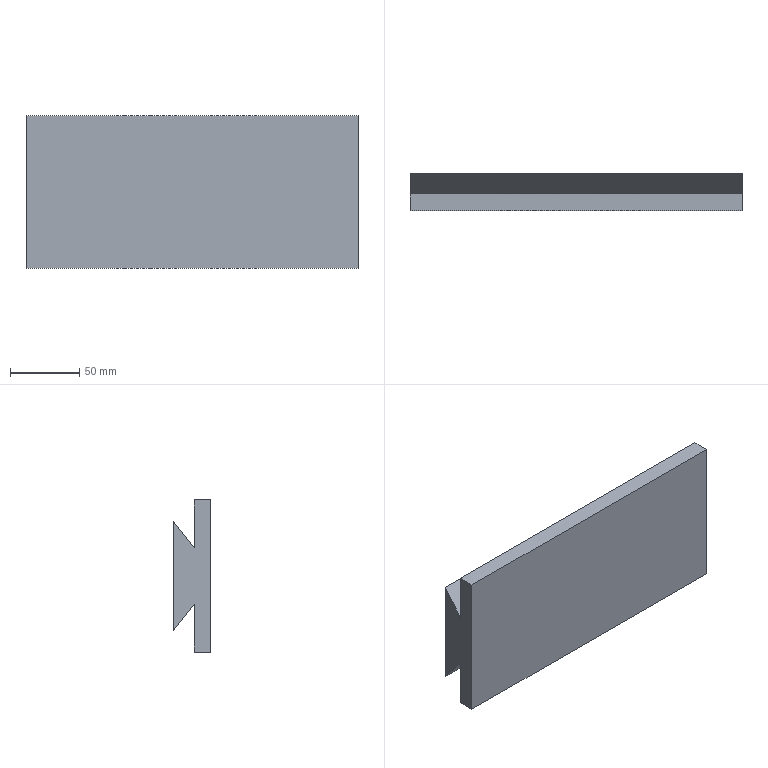Component | SolidWorks | PassiveRollerAssembly-1_DovetailPlate-1 | 1 solid | 10 faces | box 240 x 27 x 110 mm | volume 532800 mm3 | plane 10
build123d program:
from build123d import *

# Parameters (mm, degrees)
BOSS_EXTRUDE1_DEPTH = 240


with BuildPart() as part:
    # Sketch1 → Boss-Extrude1 (new body)
    with BuildSketch(Plane.XY):
        Polygon((-55, 0), (55, 0), (55, 12), (20.5, 12), (39.5, 27), (-39.5, 27), (-20.5, 12), (-55, 12), align=None)
    extrude(amount=BOSS_EXTRUDE1_DEPTH)


solid = part.part

# Placed as in the assembly
solid = solid.moved(Location((2085, 550, 270), (0, 90, 0)))
STEP:
#1=COLOUR_RGB('',0.7922,0.8196,0.9333);
#2=FILL_AREA_STYLE_COLOUR('',#1);
#3=FILL_AREA_STYLE('',(#2));
#4=SURFACE_STYLE_FILL_AREA(#3);
#5=SURFACE_SIDE_STYLE('',(#4));
#6=SURFACE_STYLE_USAGE(.BOTH.,#5);
#7=PRESENTATION_STYLE_ASSIGNMENT((#6));
#8=CARTESIAN_POINT('',(82.087,21.654,8.465));
#9=VERTEX_POINT('',#8);
#10=CARTESIAN_POINT('',(82.087,22.126,8.465));
#11=VERTEX_POINT('',#10);
#12=CARTESIAN_POINT('',(82.087,21.654,8.465));
#13=DIRECTION('',(0.,1.,-0.));
#14=VECTOR('',#13,39.37);
#15=LINE('',#12,#14);
#16=EDGE_CURVE('',#9,#11,#15,.T.);
#17=ORIENTED_EDGE('',*,*,#16,.T.);
#18=CARTESIAN_POINT('',(91.535,22.126,8.465));
#19=VERTEX_POINT('',#18);
#20=CARTESIAN_POINT('',(91.535,22.126,8.465));
#21=DIRECTION('',(-1.,0.,0.));
#22=VECTOR('',#21,39.37);
#23=LINE('',#20,#22);
#24=EDGE_CURVE('',#19,#11,#23,.T.);
#25=ORIENTED_EDGE('',*,*,#24,.F.);
#26=CARTESIAN_POINT('',(91.535,21.654,8.465));
#27=VERTEX_POINT('',#26);
#28=CARTESIAN_POINT('',(91.535,21.654,8.465));
#29=DIRECTION('',(0.,1.,-0.));
#30=VECTOR('',#29,39.37);
#31=LINE('',#28,#30);
#32=EDGE_CURVE('',#27,#19,#31,.T.);
#33=ORIENTED_EDGE('',*,*,#32,.F.);
#34=CARTESIAN_POINT('',(91.535,21.654,8.465));
#35=DIRECTION('',(-1.,0.,0.));
#36=VECTOR('',#35,39.37);
#37=LINE('',#34,#36);
#38=EDGE_CURVE('',#27,#9,#37,.T.);
#39=ORIENTED_EDGE('',*,*,#38,.T.);
#40=EDGE_LOOP('',(#17,#25,#33,#39));
#41=FACE_OUTER_BOUND('',#40,.T.);
#42=CARTESIAN_POINT('',(91.535,21.654,8.465));
#43=DIRECTION('',(0.,0.,1.));
#44=DIRECTION('',(0.,-1.,0.));
#45=AXIS2_PLACEMENT_3D('',#42,#43,#44);
#46=PLANE('',#45);
#47=ADVANCED_FACE('',(#41),#46,.F.);
#48=CARTESIAN_POINT('',(82.087,22.126,9.823));
#49=VERTEX_POINT('',#48);
#50=CARTESIAN_POINT('',(82.087,22.126,8.465));
#51=DIRECTION('',(0.,-0.,1.));
#52=VECTOR('',#51,39.37);
#53=LINE('',#50,#52);
#54=EDGE_CURVE('',#11,#49,#53,.T.);
#55=ORIENTED_EDGE('',*,*,#54,.T.);
#56=CARTESIAN_POINT('',(91.535,22.126,9.823));
#57=VERTEX_POINT('',#56);
#58=CARTESIAN_POINT('',(91.535,22.126,9.823));
#59=DIRECTION('',(-1.,0.,0.));
#60=VECTOR('',#59,39.37);
#61=LINE('',#58,#60);
#62=EDGE_CURVE('',#57,#49,#61,.T.);
#63=ORIENTED_EDGE('',*,*,#62,.F.);
#64=CARTESIAN_POINT('',(91.535,22.126,8.465));
#65=DIRECTION('',(0.,-0.,1.));
#66=VECTOR('',#65,39.37);
#67=LINE('',#64,#66);
#68=EDGE_CURVE('',#19,#57,#67,.T.);
#69=ORIENTED_EDGE('',*,*,#68,.F.);
#70=ORIENTED_EDGE('',*,*,#24,.T.);
#71=EDGE_LOOP('',(#55,#63,#69,#70));
#72=FACE_OUTER_BOUND('',#71,.T.);
#73=CARTESIAN_POINT('',(91.535,22.126,8.465));
#74=DIRECTION('',(0.,-1.,-0.));
#75=DIRECTION('',(0.,0.,-1.));
#76=AXIS2_PLACEMENT_3D('',#73,#74,#75);
#77=PLANE('',#76);
#78=ADVANCED_FACE('',(#72),#77,.F.);
#79=CARTESIAN_POINT('',(82.087,22.717,9.075));
#80=VERTEX_POINT('',#79);
#81=CARTESIAN_POINT('',(82.087,22.126,9.823));
#82=DIRECTION('',(0.,0.6196,-0.7849));
#83=VECTOR('',#82,39.37);
#84=LINE('',#81,#83);
#85=EDGE_CURVE('',#49,#80,#84,.T.);
#86=ORIENTED_EDGE('',*,*,#85,.T.);
#87=CARTESIAN_POINT('',(91.535,22.717,9.075));
#88=VERTEX_POINT('',#87);
#89=CARTESIAN_POINT('',(91.535,22.717,9.075));
#90=DIRECTION('',(-1.,0.,0.));
#91=VECTOR('',#90,39.37);
#92=LINE('',#89,#91);
#93=EDGE_CURVE('',#88,#80,#92,.T.);
#94=ORIENTED_EDGE('',*,*,#93,.F.);
#95=CARTESIAN_POINT('',(91.535,22.126,9.823));
#96=DIRECTION('',(0.,0.6196,-0.7849));
#97=VECTOR('',#96,39.37);
#98=LINE('',#95,#97);
#99=EDGE_CURVE('',#57,#88,#98,.T.);
#100=ORIENTED_EDGE('',*,*,#99,.F.);
#101=ORIENTED_EDGE('',*,*,#62,.T.);
#102=EDGE_LOOP('',(#86,#94,#100,#101));
#103=FACE_OUTER_BOUND('',#102,.T.);
#104=CARTESIAN_POINT('',(91.535,22.126,9.823));
#105=DIRECTION('',(0.,0.7849,0.6196));
#106=DIRECTION('',(0.,-0.6196,0.7849));
#107=AXIS2_PLACEMENT_3D('',#104,#105,#106);
#108=PLANE('',#107);
#109=ADVANCED_FACE('',(#103),#108,.F.);
#110=CARTESIAN_POINT('',(82.087,22.717,12.185));
#111=VERTEX_POINT('',#110);
#112=CARTESIAN_POINT('',(82.087,22.717,9.075));
#113=DIRECTION('',(0.,-0.,1.));
#114=VECTOR('',#113,39.37);
#115=LINE('',#112,#114);
#116=EDGE_CURVE('',#80,#111,#115,.T.);
#117=ORIENTED_EDGE('',*,*,#116,.T.);
#118=CARTESIAN_POINT('',(91.535,22.717,12.185));
#119=VERTEX_POINT('',#118);
#120=CARTESIAN_POINT('',(91.535,22.717,12.185));
#121=DIRECTION('',(-1.,0.,0.));
#122=VECTOR('',#121,39.37);
#123=LINE('',#120,#122);
#124=EDGE_CURVE('',#119,#111,#123,.T.);
#125=ORIENTED_EDGE('',*,*,#124,.F.);
#126=CARTESIAN_POINT('',(91.535,22.717,9.075));
#127=DIRECTION('',(0.,-0.,1.));
#128=VECTOR('',#127,39.37);
#129=LINE('',#126,#128);
#130=EDGE_CURVE('',#88,#119,#129,.T.);
#131=ORIENTED_EDGE('',*,*,#130,.F.);
#132=ORIENTED_EDGE('',*,*,#93,.T.);
#133=EDGE_LOOP('',(#117,#125,#131,#132));
#134=FACE_OUTER_BOUND('',#133,.T.);
#135=CARTESIAN_POINT('',(91.535,22.717,9.075));
#136=DIRECTION('',(0.,-1.,-0.));
#137=DIRECTION('',(0.,0.,-1.));
#138=AXIS2_PLACEMENT_3D('',#135,#136,#137);
#139=PLANE('',#138);
#140=ADVANCED_FACE('',(#134),#139,.F.);
#141=CARTESIAN_POINT('',(82.087,22.126,11.437));
#142=VERTEX_POINT('',#141);
#143=CARTESIAN_POINT('',(82.087,22.126,11.437));
#144=DIRECTION('',(0.,-0.6196,-0.7849));
#145=VECTOR('',#144,39.37);
#146=LINE('',#143,#145);
#147=EDGE_CURVE('',#111,#142,#146,.T.);
#148=ORIENTED_EDGE('',*,*,#147,.T.);
#149=CARTESIAN_POINT('',(91.535,22.126,11.437));
#150=VERTEX_POINT('',#149);
#151=CARTESIAN_POINT('',(91.535,22.126,11.437));
#152=DIRECTION('',(-1.,0.,0.));
#153=VECTOR('',#152,39.37);
#154=LINE('',#151,#153);
#155=EDGE_CURVE('',#150,#142,#154,.T.);
#156=ORIENTED_EDGE('',*,*,#155,.F.);
#157=CARTESIAN_POINT('',(91.535,22.126,11.437));
#158=DIRECTION('',(0.,-0.6196,-0.7849));
#159=VECTOR('',#158,39.37);
#160=LINE('',#157,#159);
#161=EDGE_CURVE('',#119,#150,#160,.T.);
#162=ORIENTED_EDGE('',*,*,#161,.F.);
#163=ORIENTED_EDGE('',*,*,#124,.T.);
#164=EDGE_LOOP('',(#148,#156,#162,#163));
#165=FACE_OUTER_BOUND('',#164,.T.);
#166=CARTESIAN_POINT('',(91.535,22.126,11.437));
#167=DIRECTION('',(0.,0.7849,-0.6196));
#168=DIRECTION('',(0.,0.6196,0.7849));
#169=AXIS2_PLACEMENT_3D('',#166,#167,#168);
#170=PLANE('',#169);
#171=ADVANCED_FACE('',(#165),#170,.F.);
#172=CARTESIAN_POINT('',(82.087,22.126,12.795));
#173=VERTEX_POINT('',#172);
#174=CARTESIAN_POINT('',(82.087,22.126,12.795));
#175=DIRECTION('',(0.,0.,1.));
#176=VECTOR('',#175,39.37);
#177=LINE('',#174,#176);
#178=EDGE_CURVE('',#142,#173,#177,.T.);
#179=ORIENTED_EDGE('',*,*,#178,.T.);
#180=CARTESIAN_POINT('',(91.535,22.126,12.795));
#181=VERTEX_POINT('',#180);
#182=CARTESIAN_POINT('',(91.535,22.126,12.795));
#183=DIRECTION('',(-1.,0.,0.));
#184=VECTOR('',#183,39.37);
#185=LINE('',#182,#184);
#186=EDGE_CURVE('',#181,#173,#185,.T.);
#187=ORIENTED_EDGE('',*,*,#186,.F.);
#188=CARTESIAN_POINT('',(91.535,22.126,12.795));
#189=DIRECTION('',(0.,0.,1.));
#190=VECTOR('',#189,39.37);
#191=LINE('',#188,#190);
#192=EDGE_CURVE('',#150,#181,#191,.T.);
#193=ORIENTED_EDGE('',*,*,#192,.F.);
#194=ORIENTED_EDGE('',*,*,#155,.T.);
#195=EDGE_LOOP('',(#179,#187,#193,#194));
#196=FACE_OUTER_BOUND('',#195,.T.);
#197=CARTESIAN_POINT('',(91.535,22.126,12.795));
#198=DIRECTION('',(0.,-1.,0.));
#199=DIRECTION('',(0.,-0.,-1.));
#200=AXIS2_PLACEMENT_3D('',#197,#198,#199);
#201=PLANE('',#200);
#202=ADVANCED_FACE('',(#196),#201,.F.);
#203=CARTESIAN_POINT('',(82.087,21.654,12.795));
#204=VERTEX_POINT('',#203);
#205=CARTESIAN_POINT('',(82.087,21.654,12.795));
#206=DIRECTION('',(0.,-1.,-0.));
#207=VECTOR('',#206,39.37);
#208=LINE('',#205,#207);
#209=EDGE_CURVE('',#173,#204,#208,.T.);
#210=ORIENTED_EDGE('',*,*,#209,.T.);
#211=CARTESIAN_POINT('',(91.535,21.654,12.795));
#212=VERTEX_POINT('',#211);
#213=CARTESIAN_POINT('',(91.535,21.654,12.795));
#214=DIRECTION('',(-1.,0.,0.));
#215=VECTOR('',#214,39.37);
#216=LINE('',#213,#215);
#217=EDGE_CURVE('',#212,#204,#216,.T.);
#218=ORIENTED_EDGE('',*,*,#217,.F.);
#219=CARTESIAN_POINT('',(91.535,21.654,12.795));
#220=DIRECTION('',(0.,-1.,-0.));
#221=VECTOR('',#220,39.37);
#222=LINE('',#219,#221);
#223=EDGE_CURVE('',#181,#212,#222,.T.);
#224=ORIENTED_EDGE('',*,*,#223,.F.);
#225=ORIENTED_EDGE('',*,*,#186,.T.);
#226=EDGE_LOOP('',(#210,#218,#224,#225));
#227=FACE_OUTER_BOUND('',#226,.T.);
#228=CARTESIAN_POINT('',(91.535,21.654,12.795));
#229=DIRECTION('',(0.,0.,-1.));
#230=DIRECTION('',(0.,1.,0.));
#231=AXIS2_PLACEMENT_3D('',#228,#229,#230);
#232=PLANE('',#231);
#233=ADVANCED_FACE('',(#227),#232,.F.);
#234=CARTESIAN_POINT('',(82.087,21.654,12.795));
#235=DIRECTION('',(0.,0.,-1.));
#236=VECTOR('',#235,39.37);
#237=LINE('',#234,#236);
#238=EDGE_CURVE('',#204,#9,#237,.T.);
#239=ORIENTED_EDGE('',*,*,#238,.T.);
#240=ORIENTED_EDGE('',*,*,#38,.F.);
#241=CARTESIAN_POINT('',(91.535,21.654,12.795));
#242=DIRECTION('',(0.,0.,-1.));
#243=VECTOR('',#242,39.37);
#244=LINE('',#241,#243);
#245=EDGE_CURVE('',#212,#27,#244,.T.);
#246=ORIENTED_EDGE('',*,*,#245,.F.);
#247=ORIENTED_EDGE('',*,*,#217,.T.);
#248=EDGE_LOOP('',(#239,#240,#246,#247));
#249=FACE_OUTER_BOUND('',#248,.T.);
#250=CARTESIAN_POINT('',(91.535,21.654,12.795));
#251=DIRECTION('',(0.,1.,0.));
#252=DIRECTION('',(0.,-0.,1.));
#253=AXIS2_PLACEMENT_3D('',#250,#251,#252);
#254=PLANE('',#253);
#255=ADVANCED_FACE('',(#249),#254,.F.);
#256=ORIENTED_EDGE('',*,*,#32,.T.);
#257=ORIENTED_EDGE('',*,*,#68,.T.);
#258=ORIENTED_EDGE('',*,*,#99,.T.);
#259=ORIENTED_EDGE('',*,*,#130,.T.);
#260=ORIENTED_EDGE('',*,*,#161,.T.);
#261=ORIENTED_EDGE('',*,*,#192,.T.);
#262=ORIENTED_EDGE('',*,*,#223,.T.);
#263=ORIENTED_EDGE('',*,*,#245,.T.);
#264=EDGE_LOOP('',(#256,#257,#258,#259,#260,#261,#262,#263));
#265=FACE_OUTER_BOUND('',#264,.T.);
#266=CARTESIAN_POINT('',(91.535,21.654,10.63));
#267=DIRECTION('',(1.,0.,0.));
#268=DIRECTION('',(0.,-0.,-1.));
#269=AXIS2_PLACEMENT_3D('',#266,#267,#268);
#270=PLANE('',#269);
#271=ADVANCED_FACE('',(#265),#270,.T.);
#272=ORIENTED_EDGE('',*,*,#16,.F.);
#273=ORIENTED_EDGE('',*,*,#238,.F.);
#274=ORIENTED_EDGE('',*,*,#209,.F.);
#275=ORIENTED_EDGE('',*,*,#178,.F.);
#276=ORIENTED_EDGE('',*,*,#147,.F.);
#277=ORIENTED_EDGE('',*,*,#116,.F.);
#278=ORIENTED_EDGE('',*,*,#85,.F.);
#279=ORIENTED_EDGE('',*,*,#54,.F.);
#280=EDGE_LOOP('',(#272,#273,#274,#275,#276,#277,#278,#279));
#281=FACE_OUTER_BOUND('',#280,.T.);
#282=CARTESIAN_POINT('',(82.087,21.654,10.63));
#283=DIRECTION('',(1.,0.,0.));
#284=DIRECTION('',(0.,-0.,-1.));
#285=AXIS2_PLACEMENT_3D('',#282,#283,#284);
#286=PLANE('',#285);
#287=ADVANCED_FACE('',(#281),#286,.F.);
#288=CLOSED_SHELL('',(#47,#78,#109,#140,#171,#202,#233,#255,#271,#287));
#289=MANIFOLD_SOLID_BREP('',#288);
#290=STYLED_ITEM('',(#7),#289);
#291=(LENGTH_UNIT()NAMED_UNIT(*)SI_UNIT($,.METRE.));
#292=LENGTH_MEASURE_WITH_UNIT(LENGTH_MEASURE(0.0254),#291);
#293=DIMENSIONAL_EXPONENTS(1.,0.,0.,0.,0.,0.,0.);
#294=(CONVERSION_BASED_UNIT('',#292)LENGTH_UNIT()NAMED_UNIT(#293));
#295=UNCERTAINTY_MEASURE_WITH_UNIT(LENGTH_MEASURE(0.00001),#294,'','');
#296=(NAMED_UNIT(*)PLANE_ANGLE_UNIT()SI_UNIT($,.RADIAN.));
#297=(NAMED_UNIT(*)SI_UNIT($,.STERADIAN.)SOLID_ANGLE_UNIT());
#298=(GEOMETRIC_REPRESENTATION_CONTEXT(3)GLOBAL_UNCERTAINTY_ASSIGNED_CONTEXT((#295))GLOBAL_UNIT_ASSIGNED_CONTEXT((#294,#296,#297))REPRESENTATION_CONTEXT('',''));
#299=MECHANICAL_DESIGN_GEOMETRIC_PRESENTATION_REPRESENTATION('',(#290),#298);
#300=CARTESIAN_POINT('',(0.,0.,0.));
#301=DIRECTION('',(0.,0.,1.));
#302=DIRECTION('',(1.,0.,0.));
#303=AXIS2_PLACEMENT_3D('',#300,#301,#302);
#304=(LENGTH_UNIT()NAMED_UNIT(*)SI_UNIT($,.METRE.));
#305=LENGTH_MEASURE_WITH_UNIT(LENGTH_MEASURE(0.0254),#304);
#306=DIMENSIONAL_EXPONENTS(1.,0.,0.,0.,0.,0.,0.);
#307=(CONVERSION_BASED_UNIT('',#305)LENGTH_UNIT()NAMED_UNIT(#306));
#308=UNCERTAINTY_MEASURE_WITH_UNIT(LENGTH_MEASURE(0.00001),#307,'','');
#309=(NAMED_UNIT(*)PLANE_ANGLE_UNIT()SI_UNIT($,.RADIAN.));
#310=(NAMED_UNIT(*)SI_UNIT($,.STERADIAN.)SOLID_ANGLE_UNIT());
#311=(GEOMETRIC_REPRESENTATION_CONTEXT(3)GLOBAL_UNCERTAINTY_ASSIGNED_CONTEXT((#308))GLOBAL_UNIT_ASSIGNED_CONTEXT((#307,#309,#310))REPRESENTATION_CONTEXT('',''));
#312=ADVANCED_BREP_SHAPE_REPRESENTATION('',(#289,#303),#311);
#313=PRESENTATION_LAYER_ASSIGNMENT('','',(#290));